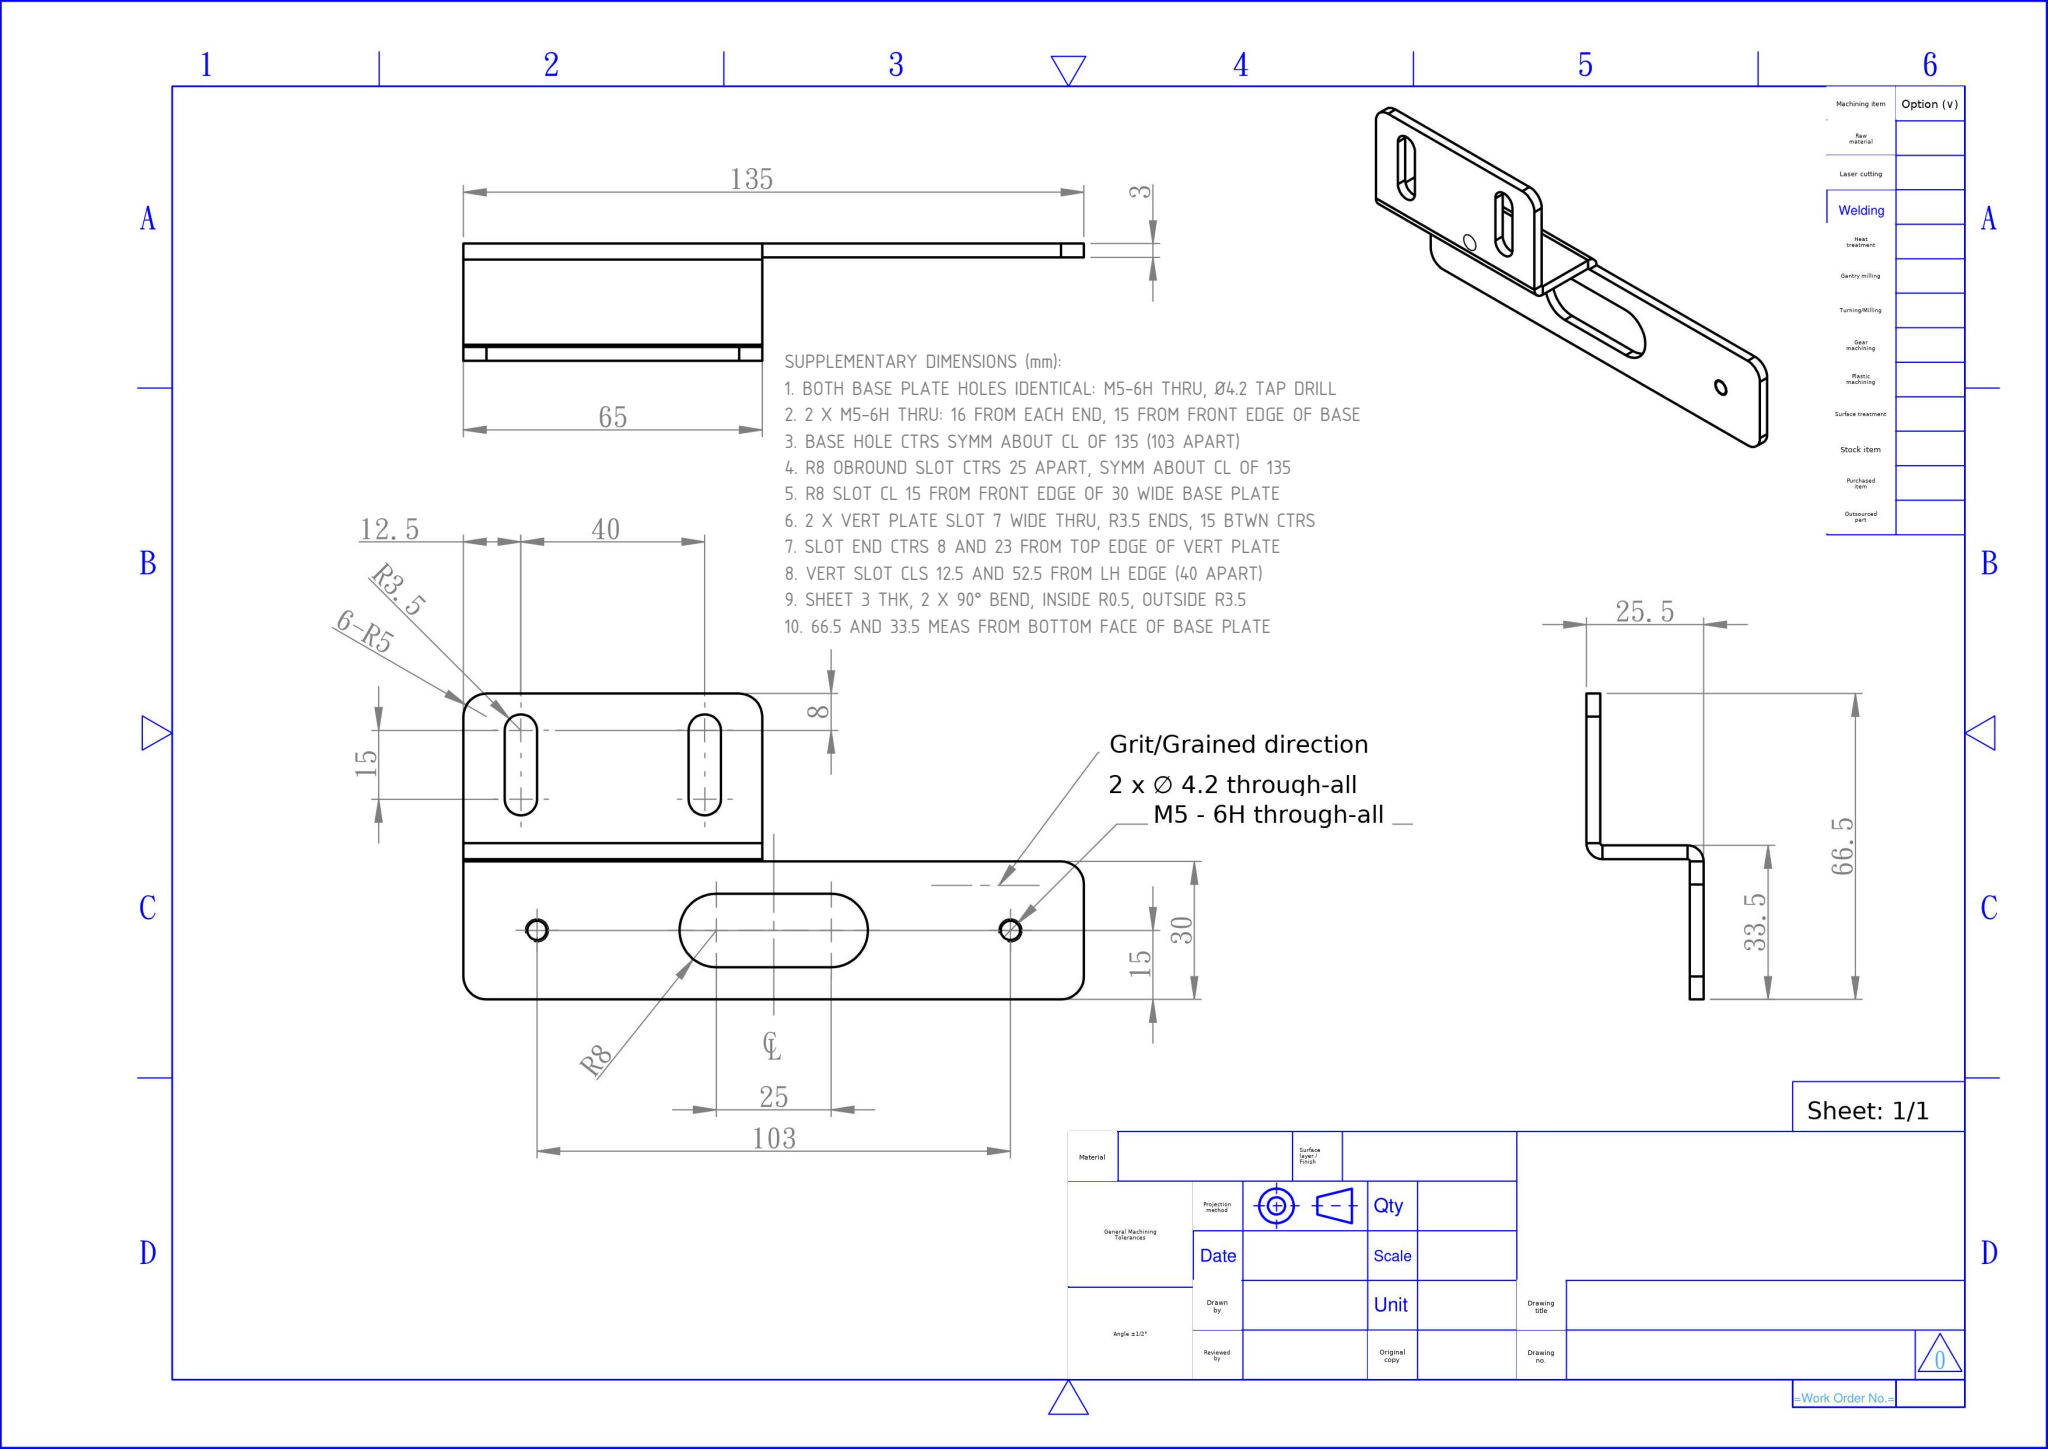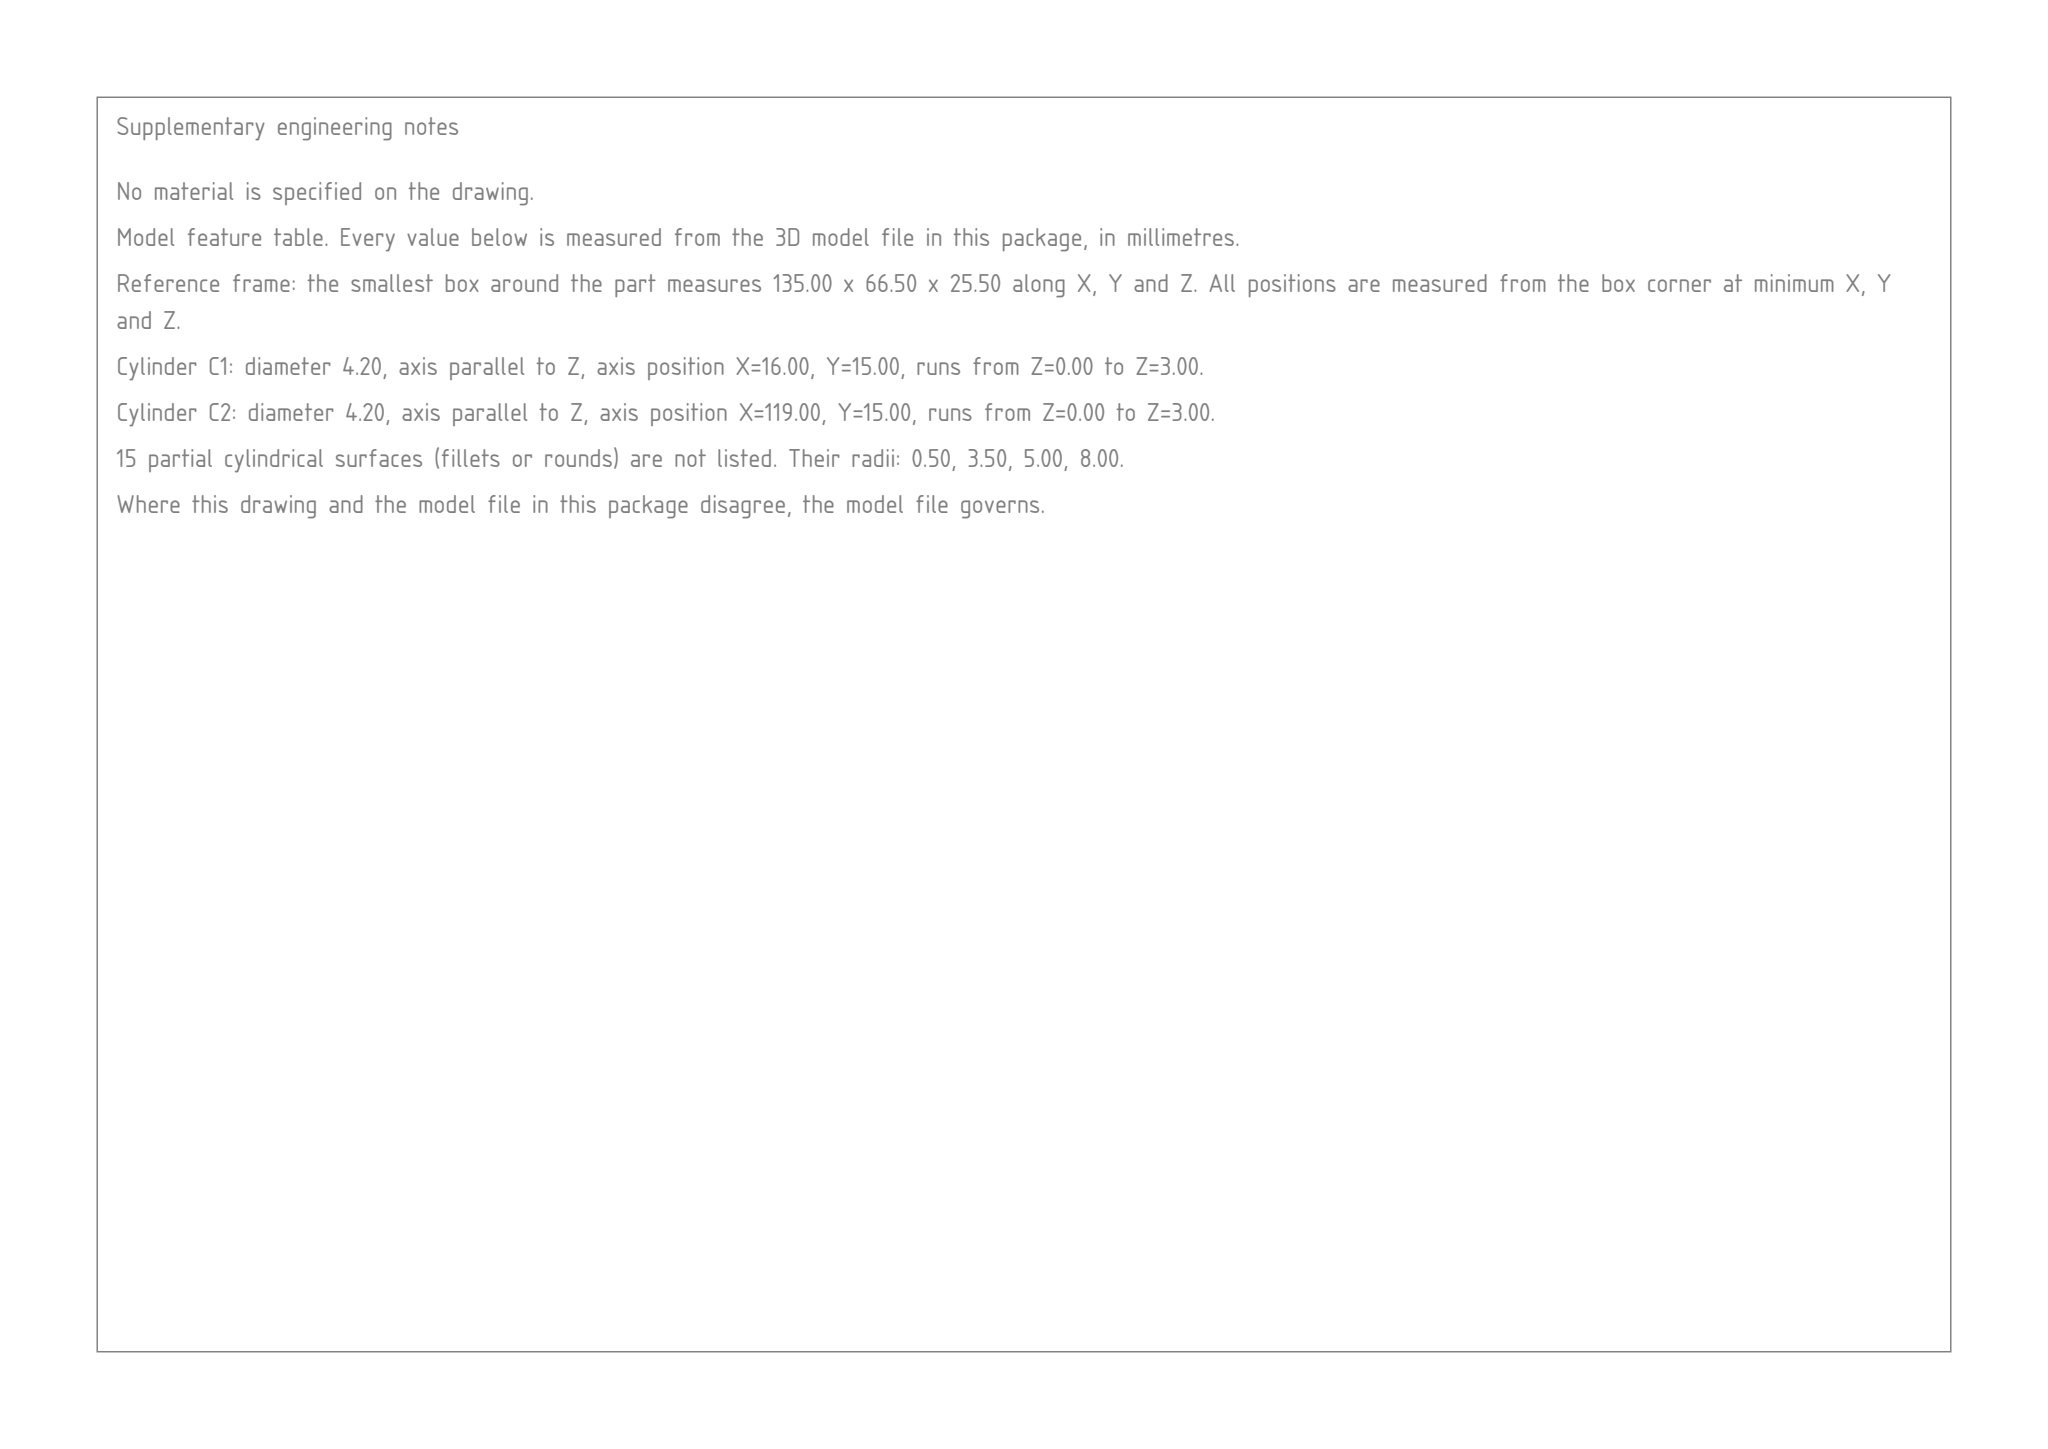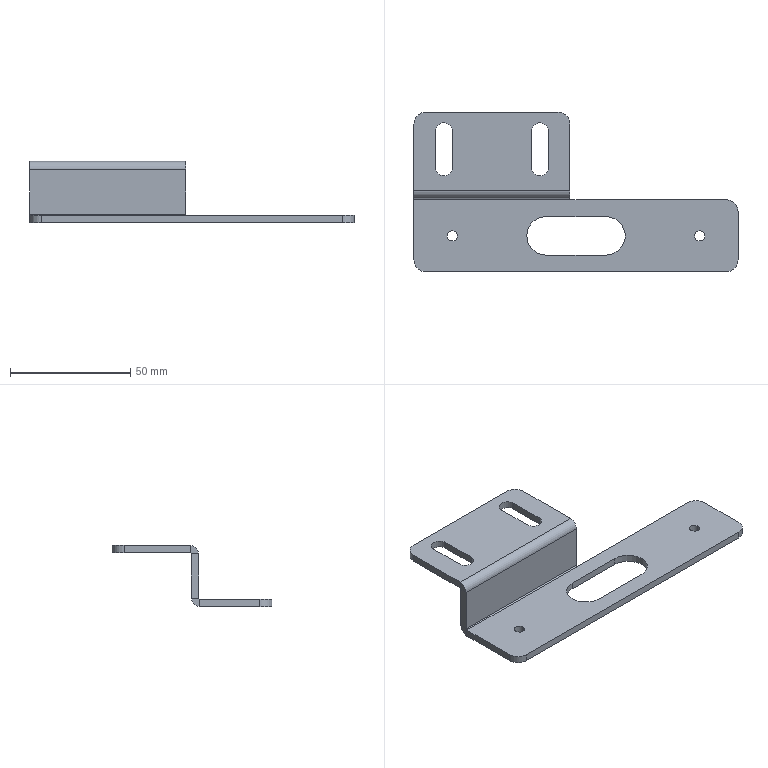Part | SolidWorks | mm | 1 solid | 45 faces | box 135 x 66.5 x 25.5 mm | volume 20493 mm3 | plane 25 | cylinder 20 | commonest cylinder face diameters 7 x6 10 x5 4.2 x4 16 x3 1 x2